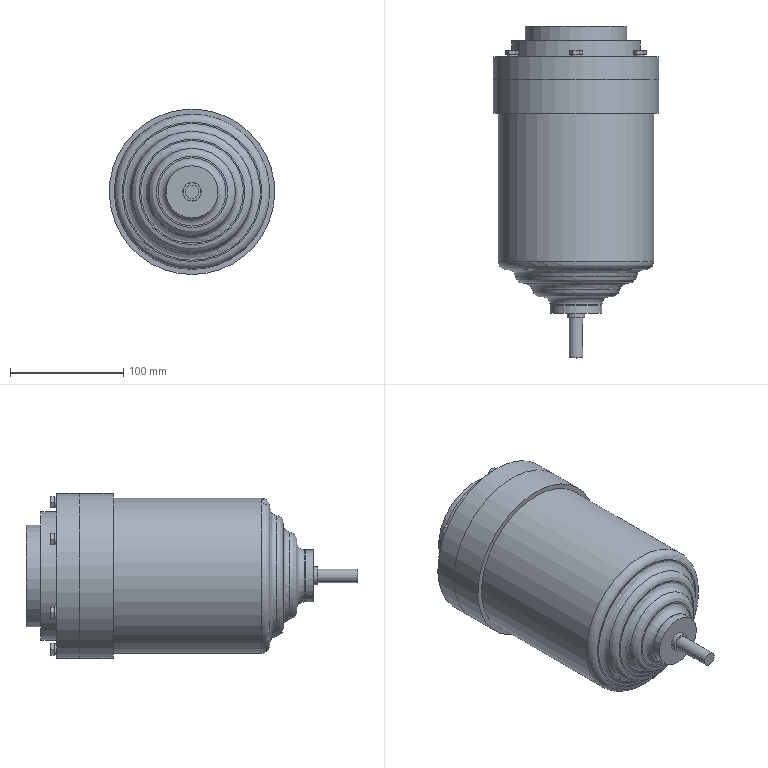Assembly | NX | mm | 37 component files | 55 solids | 558 faces | box 146 x 293 x 146 mm | volume 2402974 mm3 | plane 239 | cylinder 140 | cone 102 | spline 30 | torus 25 | sphere 22 | commonest cylinder face diameters 20 x12 8 x12 16 x8 12 x7 6 x6 9.88 x6 6.68 x6 8.74 x6
Bill of materials:
GB-T5782-2000,M6x30 | 6 |  | Hexagon Head Bolt, GB-T 5782-2000,M6x30
unnamed part 1 | 1 |  | Thin flat annular disc (plain washer-like ring) with a single central through hole.
unnamed part 2 | 6 |  | Solid cylindrical rod/pin with one hemispherical (domed) end and one flat end.
unnamed part 3 | 1 |  | Stepped circular flange/hub disc: a wide central flange with smaller-diameter coaxial steps on both sides, a bolt-circle of through holes, multiple smaller conical-bottom holes, and a central bore with internal groove opening on one face.
unnamed part 4 | 1 |  | Flanged cylindrical bushing/sleeve: hollow cylinder with a short larger-diameter collar at one end and a central through bore.
unnamed part 5 | 1 |  | Thick annular ring/spacer with a large central through hole relative to its outer diameter.
GB-T292_AC-1994,7203_AC | 2 |  | Annular assembly-like body resembling an open radial ball bearing: a thin outer ring and an inner ring with a central through-bore, with eight spherical rolling elements evenly spaced in the annular gap between the rings.
GB93-87,6 | 6 |  | Single Coil Spring Lock Washer, Normal Type, GB 93-87,6
GB-T70.1-2000,M5x12 | 4 |  | Hexagon Socket Head Cap Screw, GB-T 70.1-2000,M5x12
unnamed part 6 | 1 |  | Stepped shaft with a coaxial larger cylindrical body (rotor/drum-like) carrying six axial holes on a circle; the shaft extends a long distance from one side with several diameter steps and a short distance from the other.
unnamed part 7 | 6 |  | Helical coil spring of round wire with about ten open-pitch coils of constant diameter; open-coil form looks like a compression spring.
unnamed part 8 | 1 |  | Cup or cap-shaped body of revolution: main cylindrical body with a slightly larger rim/collar at one end, and at the other end a stepped, tapering series of concentric shoulders ending in a small central through hole.
unnamed part 9 | 1 |  | Thin flat circular plate/disc with a large central through hole, six medium through holes on an inner circle, and four small through holes near the outer edge.
Mates:
1. concentric | port_plate 1 edge | cover 1 edge
2. concentric | rotor 1 edge | port_plate 1 edge
3. concentric | housing 1 edge | cover 1 edge
4. concentric | bushing 1 edge | housing 1 edge
5. fix | cover 1 component
6. concentric | bearing 2 edge | cover 1 edge
7. concentric | bearing 1 edge | housing 1 edge
8. concentric | oil_seal 1 edge | bushing 1 edge
9. concentric | spring_washer_M6 6 edge | cover 1 edge
10. concentric | bolt_M6x30 6 edge | spring_washer_M6 6 edge
11. bond | cover 1 component | assembly component
12. bond | spring_washer_M6 6 component | assembly component
13. bond | bolt_M6x30 6 component | assembly component
14. bond | spring_washer_M6 5 component | assembly component
15. bond | bolt_M6x30 5 component | assembly component
16. bond | spring_washer_M6 4 component | assembly component
17. bond | bolt_M6x30 4 component | assembly component
18. bond | spring_washer_M6 3 component | assembly component
19. bond | bolt_M6x30 3 component | assembly component
20. bond | spring_washer_M6 2 component | assembly component
21. bond | bolt_M6x30 2 component | assembly component
22. bond | spring_washer_M6 1 component | assembly component
23. bond | bolt_M6x30 1 component | assembly component
24. circular | assembly datumaxis | assembly cartesiancoordinatesystem | assembly cartesiancoordinatesystem | assembly cartesiancoordinatesystem | assembly cartesiancoordinatesystem | assembly cartesiancoordinatesystem | assembly cartesiancoordinatesystem
25. circular | assembly datumaxis | assembly cartesiancoordinatesystem | assembly cartesiancoordinatesystem | assembly cartesiancoordinatesystem | assembly cartesiancoordinatesystem | assembly cartesiancoordinatesystem | assembly cartesiancoordinatesystem
26. concentric | screw_M5x12 4 edge | port_plate 1 edge
27. bond | housing 1 component | assembly component
28. bond | screw_M5x12 4 component | assembly component
29. bond | screw_M5x12 3 component | assembly component
30. bond | screw_M5x12 2 component | assembly component
31. bond | screw_M5x12 1 component | assembly component
32. circular | assembly datumaxis | assembly cartesiancoordinatesystem | assembly cartesiancoordinatesystem | assembly cartesiancoordinatesystem | assembly cartesiancoordinatesystem
33. touch align | plunger 6 face | rotor 1 face
34. distance | plunger 6 face | rotor 1 face
35. bond | rotor 1 component | assembly component
36. bond | plunger 6 component | assembly component
37. bond | plunger 5 component | assembly component
38. bond | plunger 4 component | assembly component
39. bond | plunger 3 component | assembly component
40. circular | assembly datumaxis | assembly cartesiancoordinatesystem | assembly cartesiancoordinatesystem | assembly cartesiancoordinatesystem | assembly cartesiancoordinatesystem | assembly cartesiancoordinatesystem | assembly cartesiancoordinatesystem
41. bond | plunger 2 component | assembly component
42. bond | plunger 1 component | assembly component
43. touch align | swash_plate 1 face | housing 1 face
44. touch align | swash_plate 1 face | plunger 6 face
45. concentric | spring 6 edge | rotor 1 edge
46. bond | rotor 1 component | assembly component
47. bond | spring 6 component | assembly component
48. bond | spring 5 component | assembly component
49. bond | spring 4 component | assembly component
50. bond | spring 3 component | assembly component
51. bond | spring 2 component | assembly component
52. bond | spring 1 component | assembly component
53. circular | assembly datumaxis | assembly cartesiancoordinatesystem | assembly cartesiancoordinatesystem | assembly cartesiancoordinatesystem | assembly cartesiancoordinatesystem | assembly cartesiancoordinatesystem | assembly cartesiancoordinatesystem